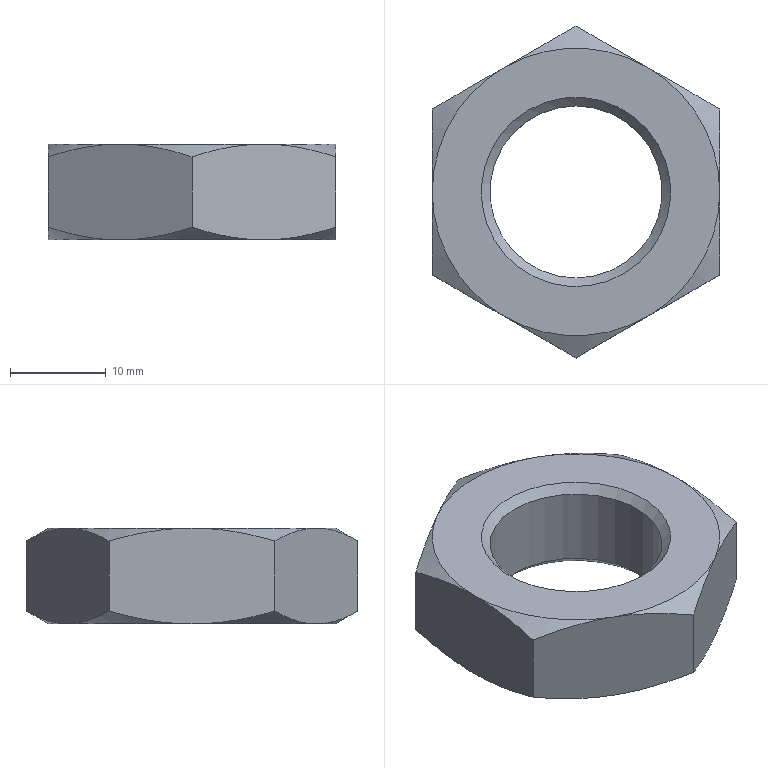Component | NX | GB-T6172_1-2000_M20X2_5_2 | 1 solid | 23 faces | volume 5151 mm3 | cone 14 | plane 8 | cylinder 1 | commonest cylinder face diameters 17.97 x1